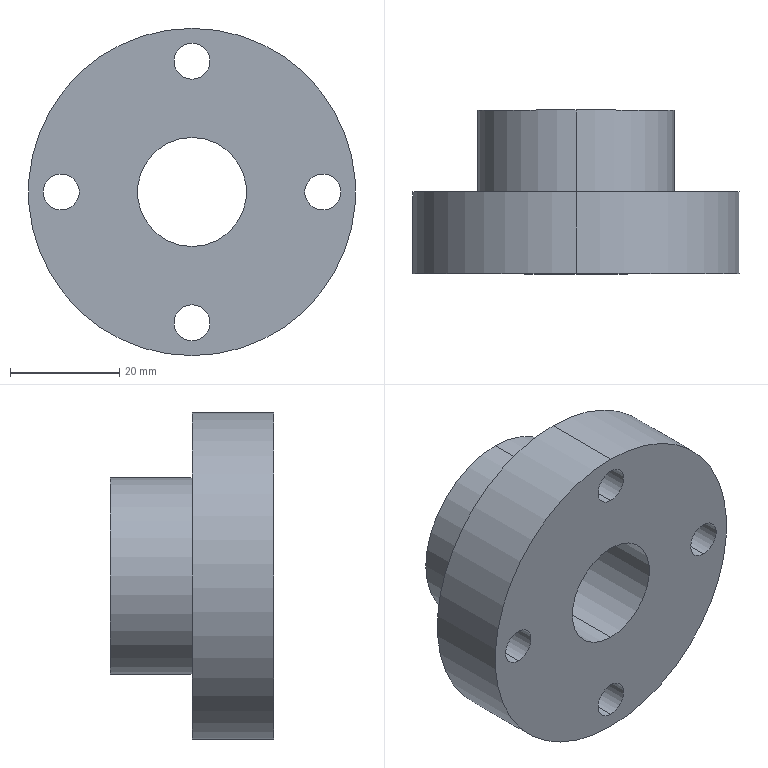Component | SolidWorks | OpticalAxisSeat1-1-1 | 1 solid | 29 faces | box 60 x 30 x 60 mm | volume 44996 mm3 | cylinder 22 | plane 7 | commonest cylinder face diameters 10 x8 6.6 x8 36 x2 60 x2 20 x2
build123d program:
from build123d import *

# Parameters (mm, degrees)
HOLE_SIZE_ACCORDING_TO_TYPE_1_OF_HEXAG_D           = 6.6
HOLE_SIZE_ACCORDING_TO_TYPE_1_OF_HEXAG_CBORE_D     = 10
HOLE_SIZE_ACCORDING_TO_TYPE_1_OF_HEXAG_CBORE_DEPTH = 6.8
CIRPATTERN1_COUNT                                  = 4


with BuildPart() as part:
    # Sketch1 → Revolve1 (revolve)
    with BuildSketch(Plane.XY, mode=Mode.PRIVATE) as revolve1_sk:
        Polygon((10, 1.22), (30, 1.22), (30, 16.22), (18, 16.22), (18, 31.22), (10, 31.22), align=None)
    revolve(revolve1_sk.sketch.rotate(Axis((0, 0, 0), (0, 1, 0)), 90), axis=Axis((0, 0, 0), (0, 1, 0)))

    # Hole Size _According to_ Type 1 of Hexag (through all)
    with Locations(Plane(origin=(24, 16.22, 0), x_dir=(0, 0, 1), z_dir=(0, 1, 0))):
        with Locations((0, 0)):
            hole_size_according_to_type_1_of_hexag = CounterBoreHole(HOLE_SIZE_ACCORDING_TO_TYPE_1_OF_HEXAG_D / 2, HOLE_SIZE_ACCORDING_TO_TYPE_1_OF_HEXAG_CBORE_D / 2, HOLE_SIZE_ACCORDING_TO_TYPE_1_OF_HEXAG_CBORE_DEPTH)

    # CirPattern1: Hole Size _According to_ Type 1 of Hexag ×4 about axis
    cirpattern1_axis = Axis((0, 0, 0), (0, 1, 0))
    for i in range(1, CIRPATTERN1_COUNT):
        add(hole_size_according_to_type_1_of_hexag.rotate(cirpattern1_axis, i * 360 / CIRPATTERN1_COUNT), mode=Mode.SUBTRACT)


solid = part.part

# Placed as in the assembly
solid = solid.moved(Location((-30.965, -1.22, 663.073), (0, 0, 0)))
STEP:
#1=CARTESIAN_POINT('',(-1.219,0.3228,24.964));
#2=VERTEX_POINT('',#1);
#3=CARTESIAN_POINT('',(-1.219,0.3228,25.357));
#4=VERTEX_POINT('',#3);
#5=CARTESIAN_POINT('',(-1.219,0.3228,25.16));
#6=DIRECTION('',(0.,1.,0.));
#7=DIRECTION('',(0.,0.,1.));
#8=AXIS2_PLACEMENT_3D('',#5,#6,#7);
#9=CIRCLE('',#8,0.1969);
#10=EDGE_CURVE('',#2,#4,#9,.T.);
#11=ORIENTED_EDGE('',*,*,#10,.F.);
#12=CARTESIAN_POINT('',(-1.219,0.5906,24.964));
#13=VERTEX_POINT('',#12);
#14=CARTESIAN_POINT('',(-1.219,0.5906,24.964));
#15=DIRECTION('',(0.,1.,0.));
#16=VECTOR('',#15,39.37);
#17=LINE('',#14,#16);
#18=EDGE_CURVE('',#2,#13,#17,.T.);
#19=ORIENTED_EDGE('',*,*,#18,.T.);
#20=CARTESIAN_POINT('',(-1.219,0.5906,25.357));
#21=VERTEX_POINT('',#20);
#22=CARTESIAN_POINT('',(-1.219,0.5906,25.16));
#23=DIRECTION('',(0.,1.,0.));
#24=DIRECTION('',(0.,0.,1.));
#25=AXIS2_PLACEMENT_3D('',#22,#23,#24);
#26=CIRCLE('',#25,0.1969);
#27=EDGE_CURVE('',#13,#21,#26,.T.);
#28=ORIENTED_EDGE('',*,*,#27,.T.);
#29=CARTESIAN_POINT('',(-1.219,0.5906,25.357));
#30=DIRECTION('',(0.,1.,0.));
#31=VECTOR('',#30,39.37);
#32=LINE('',#29,#31);
#33=EDGE_CURVE('',#4,#21,#32,.T.);
#34=ORIENTED_EDGE('',*,*,#33,.F.);
#35=EDGE_LOOP('',(#11,#19,#28,#34));
#36=FACE_OUTER_BOUND('',#35,.T.);
#37=CARTESIAN_POINT('',(-1.219,0.5906,25.16));
#38=DIRECTION('',(0.,1.,0.));
#39=DIRECTION('',(0.,0.,1.));
#40=AXIS2_PLACEMENT_3D('',#37,#38,#39);
#41=CYLINDRICAL_SURFACE('',#40,0.1969);
#42=ADVANCED_FACE('',(#36),#41,.F.);
#43=CARTESIAN_POINT('',(-1.219,-0.,25.03));
#44=VERTEX_POINT('',#43);
#45=CARTESIAN_POINT('',(-1.219,-0.,25.29));
#46=VERTEX_POINT('',#45);
#47=CARTESIAN_POINT('',(-1.219,-0.,25.16));
#48=DIRECTION('',(0.,1.,0.));
#49=DIRECTION('',(0.,0.,1.));
#50=AXIS2_PLACEMENT_3D('',#47,#48,#49);
#51=CIRCLE('',#50,0.1299);
#52=EDGE_CURVE('',#44,#46,#51,.T.);
#53=ORIENTED_EDGE('',*,*,#52,.F.);
#54=CARTESIAN_POINT('',(-1.219,0.3228,25.03));
#55=VERTEX_POINT('',#54);
#56=CARTESIAN_POINT('',(-1.219,0.5906,25.03));
#57=DIRECTION('',(0.,1.,0.));
#58=VECTOR('',#57,39.37);
#59=LINE('',#56,#58);
#60=EDGE_CURVE('',#44,#55,#59,.T.);
#61=ORIENTED_EDGE('',*,*,#60,.T.);
#62=CARTESIAN_POINT('',(-1.219,0.3228,25.29));
#63=VERTEX_POINT('',#62);
#64=CARTESIAN_POINT('',(-1.219,0.3228,25.16));
#65=DIRECTION('',(0.,1.,0.));
#66=DIRECTION('',(0.,0.,1.));
#67=AXIS2_PLACEMENT_3D('',#64,#65,#66);
#68=CIRCLE('',#67,0.1299);
#69=EDGE_CURVE('',#55,#63,#68,.T.);
#70=ORIENTED_EDGE('',*,*,#69,.T.);
#71=CARTESIAN_POINT('',(-1.219,0.5906,25.29));
#72=DIRECTION('',(0.,1.,0.));
#73=VECTOR('',#72,39.37);
#74=LINE('',#71,#73);
#75=EDGE_CURVE('',#46,#63,#74,.T.);
#76=ORIENTED_EDGE('',*,*,#75,.F.);
#77=EDGE_LOOP('',(#53,#61,#70,#76));
#78=FACE_OUTER_BOUND('',#77,.T.);
#79=CARTESIAN_POINT('',(-1.219,0.5906,25.16));
#80=DIRECTION('',(0.,1.,0.));
#81=DIRECTION('',(0.,0.,1.));
#82=AXIS2_PLACEMENT_3D('',#79,#80,#81);
#83=CYLINDRICAL_SURFACE('',#82,0.1299);
#84=ADVANCED_FACE('',(#78),#83,.F.);
#85=CARTESIAN_POINT('',(-2.164,0.3228,25.908));
#86=VERTEX_POINT('',#85);
#87=CARTESIAN_POINT('',(-2.164,0.3228,26.302));
#88=VERTEX_POINT('',#87);
#89=CARTESIAN_POINT('',(-2.164,0.3228,26.105));
#90=DIRECTION('',(0.,1.,0.));
#91=DIRECTION('',(0.,0.,1.));
#92=AXIS2_PLACEMENT_3D('',#89,#90,#91);
#93=CIRCLE('',#92,0.1969);
#94=EDGE_CURVE('',#86,#88,#93,.T.);
#95=ORIENTED_EDGE('',*,*,#94,.F.);
#96=CARTESIAN_POINT('',(-2.164,0.5906,25.908));
#97=VERTEX_POINT('',#96);
#98=CARTESIAN_POINT('',(-2.164,0.5906,25.908));
#99=DIRECTION('',(0.,1.,0.));
#100=VECTOR('',#99,39.37);
#101=LINE('',#98,#100);
#102=EDGE_CURVE('',#86,#97,#101,.T.);
#103=ORIENTED_EDGE('',*,*,#102,.T.);
#104=CARTESIAN_POINT('',(-2.164,0.5906,26.302));
#105=VERTEX_POINT('',#104);
#106=CARTESIAN_POINT('',(-2.164,0.5906,26.105));
#107=DIRECTION('',(0.,1.,0.));
#108=DIRECTION('',(0.,0.,1.));
#109=AXIS2_PLACEMENT_3D('',#106,#107,#108);
#110=CIRCLE('',#109,0.1969);
#111=EDGE_CURVE('',#97,#105,#110,.T.);
#112=ORIENTED_EDGE('',*,*,#111,.T.);
#113=CARTESIAN_POINT('',(-2.164,0.5906,26.302));
#114=DIRECTION('',(0.,1.,0.));
#115=VECTOR('',#114,39.37);
#116=LINE('',#113,#115);
#117=EDGE_CURVE('',#88,#105,#116,.T.);
#118=ORIENTED_EDGE('',*,*,#117,.F.);
#119=EDGE_LOOP('',(#95,#103,#112,#118));
#120=FACE_OUTER_BOUND('',#119,.T.);
#121=CARTESIAN_POINT('',(-2.164,0.5906,26.105));
#122=DIRECTION('',(0.,1.,0.));
#123=DIRECTION('',(0.,0.,1.));
#124=AXIS2_PLACEMENT_3D('',#121,#122,#123);
#125=CYLINDRICAL_SURFACE('',#124,0.1969);
#126=ADVANCED_FACE('',(#120),#125,.F.);
#127=CARTESIAN_POINT('',(-2.164,-0.,25.975));
#128=VERTEX_POINT('',#127);
#129=CARTESIAN_POINT('',(-2.164,-0.,26.235));
#130=VERTEX_POINT('',#129);
#131=CARTESIAN_POINT('',(-2.164,-0.,26.105));
#132=DIRECTION('',(0.,1.,0.));
#133=DIRECTION('',(0.,0.,1.));
#134=AXIS2_PLACEMENT_3D('',#131,#132,#133);
#135=CIRCLE('',#134,0.1299);
#136=EDGE_CURVE('',#128,#130,#135,.T.);
#137=ORIENTED_EDGE('',*,*,#136,.F.);
#138=CARTESIAN_POINT('',(-2.164,0.3228,25.975));
#139=VERTEX_POINT('',#138);
#140=CARTESIAN_POINT('',(-2.164,0.5906,25.975));
#141=DIRECTION('',(0.,1.,0.));
#142=VECTOR('',#141,39.37);
#143=LINE('',#140,#142);
#144=EDGE_CURVE('',#128,#139,#143,.T.);
#145=ORIENTED_EDGE('',*,*,#144,.T.);
#146=CARTESIAN_POINT('',(-2.164,0.3228,26.235));
#147=VERTEX_POINT('',#146);
#148=CARTESIAN_POINT('',(-2.164,0.3228,26.105));
#149=DIRECTION('',(0.,1.,0.));
#150=DIRECTION('',(0.,0.,1.));
#151=AXIS2_PLACEMENT_3D('',#148,#149,#150);
#152=CIRCLE('',#151,0.1299);
#153=EDGE_CURVE('',#139,#147,#152,.T.);
#154=ORIENTED_EDGE('',*,*,#153,.T.);
#155=CARTESIAN_POINT('',(-2.164,0.5906,26.235));
#156=DIRECTION('',(0.,1.,0.));
#157=VECTOR('',#156,39.37);
#158=LINE('',#155,#157);
#159=EDGE_CURVE('',#130,#147,#158,.T.);
#160=ORIENTED_EDGE('',*,*,#159,.F.);
#161=EDGE_LOOP('',(#137,#145,#154,#160));
#162=FACE_OUTER_BOUND('',#161,.T.);
#163=CARTESIAN_POINT('',(-2.164,0.5906,26.105));
#164=DIRECTION('',(0.,1.,0.));
#165=DIRECTION('',(0.,0.,1.));
#166=AXIS2_PLACEMENT_3D('',#163,#164,#165);
#167=CYLINDRICAL_SURFACE('',#166,0.1299);
#168=ADVANCED_FACE('',(#162),#167,.F.);
#169=CARTESIAN_POINT('',(-1.219,0.3228,26.853));
#170=VERTEX_POINT('',#169);
#171=CARTESIAN_POINT('',(-1.219,0.3228,27.247));
#172=VERTEX_POINT('',#171);
#173=CARTESIAN_POINT('',(-1.219,0.3228,27.05));
#174=DIRECTION('',(0.,1.,0.));
#175=DIRECTION('',(0.,0.,1.));
#176=AXIS2_PLACEMENT_3D('',#173,#174,#175);
#177=CIRCLE('',#176,0.1969);
#178=EDGE_CURVE('',#170,#172,#177,.T.);
#179=ORIENTED_EDGE('',*,*,#178,.F.);
#180=CARTESIAN_POINT('',(-1.219,0.5906,26.853));
#181=VERTEX_POINT('',#180);
#182=CARTESIAN_POINT('',(-1.219,0.5906,26.853));
#183=DIRECTION('',(0.,1.,0.));
#184=VECTOR('',#183,39.37);
#185=LINE('',#182,#184);
#186=EDGE_CURVE('',#170,#181,#185,.T.);
#187=ORIENTED_EDGE('',*,*,#186,.T.);
#188=CARTESIAN_POINT('',(-1.219,0.5906,27.247));
#189=VERTEX_POINT('',#188);
#190=CARTESIAN_POINT('',(-1.219,0.5906,27.05));
#191=DIRECTION('',(0.,1.,0.));
#192=DIRECTION('',(0.,0.,1.));
#193=AXIS2_PLACEMENT_3D('',#190,#191,#192);
#194=CIRCLE('',#193,0.1969);
#195=EDGE_CURVE('',#181,#189,#194,.T.);
#196=ORIENTED_EDGE('',*,*,#195,.T.);
#197=CARTESIAN_POINT('',(-1.219,0.5906,27.247));
#198=DIRECTION('',(0.,1.,0.));
#199=VECTOR('',#198,39.37);
#200=LINE('',#197,#199);
#201=EDGE_CURVE('',#172,#189,#200,.T.);
#202=ORIENTED_EDGE('',*,*,#201,.F.);
#203=EDGE_LOOP('',(#179,#187,#196,#202));
#204=FACE_OUTER_BOUND('',#203,.T.);
#205=CARTESIAN_POINT('',(-1.219,0.5906,27.05));
#206=DIRECTION('',(0.,1.,0.));
#207=DIRECTION('',(0.,0.,1.));
#208=AXIS2_PLACEMENT_3D('',#205,#206,#207);
#209=CYLINDRICAL_SURFACE('',#208,0.1969);
#210=ADVANCED_FACE('',(#204),#209,.F.);
#211=CARTESIAN_POINT('',(-1.219,-0.,26.92));
#212=VERTEX_POINT('',#211);
#213=CARTESIAN_POINT('',(-1.219,-0.,27.18));
#214=VERTEX_POINT('',#213);
#215=CARTESIAN_POINT('',(-1.219,-0.,27.05));
#216=DIRECTION('',(0.,1.,0.));
#217=DIRECTION('',(0.,0.,1.));
#218=AXIS2_PLACEMENT_3D('',#215,#216,#217);
#219=CIRCLE('',#218,0.1299);
#220=EDGE_CURVE('',#212,#214,#219,.T.);
#221=ORIENTED_EDGE('',*,*,#220,.F.);
#222=CARTESIAN_POINT('',(-1.219,0.3228,26.92));
#223=VERTEX_POINT('',#222);
#224=CARTESIAN_POINT('',(-1.219,0.5906,26.92));
#225=DIRECTION('',(0.,1.,0.));
#226=VECTOR('',#225,39.37);
#227=LINE('',#224,#226);
#228=EDGE_CURVE('',#212,#223,#227,.T.);
#229=ORIENTED_EDGE('',*,*,#228,.T.);
#230=CARTESIAN_POINT('',(-1.219,0.3228,27.18));
#231=VERTEX_POINT('',#230);
#232=CARTESIAN_POINT('',(-1.219,0.3228,27.05));
#233=DIRECTION('',(0.,1.,0.));
#234=DIRECTION('',(0.,0.,1.));
#235=AXIS2_PLACEMENT_3D('',#232,#233,#234);
#236=CIRCLE('',#235,0.1299);
#237=EDGE_CURVE('',#223,#231,#236,.T.);
#238=ORIENTED_EDGE('',*,*,#237,.T.);
#239=CARTESIAN_POINT('',(-1.219,0.5906,27.18));
#240=DIRECTION('',(0.,1.,0.));
#241=VECTOR('',#240,39.37);
#242=LINE('',#239,#241);
#243=EDGE_CURVE('',#214,#231,#242,.T.);
#244=ORIENTED_EDGE('',*,*,#243,.F.);
#245=EDGE_LOOP('',(#221,#229,#238,#244));
#246=FACE_OUTER_BOUND('',#245,.T.);
#247=CARTESIAN_POINT('',(-1.219,0.5906,27.05));
#248=DIRECTION('',(0.,1.,0.));
#249=DIRECTION('',(0.,0.,1.));
#250=AXIS2_PLACEMENT_3D('',#247,#248,#249);
#251=CYLINDRICAL_SURFACE('',#250,0.1299);
#252=ADVANCED_FACE('',(#246),#251,.F.);
#253=CARTESIAN_POINT('',(-0.2742,0.3228,25.908));
#254=VERTEX_POINT('',#253);
#255=CARTESIAN_POINT('',(-0.2742,0.3228,26.302));
#256=VERTEX_POINT('',#255);
#257=CARTESIAN_POINT('',(-0.2742,0.3228,26.105));
#258=DIRECTION('',(0.,1.,0.));
#259=DIRECTION('',(0.,0.,1.));
#260=AXIS2_PLACEMENT_3D('',#257,#258,#259);
#261=CIRCLE('',#260,0.1969);
#262=EDGE_CURVE('',#254,#256,#261,.T.);
#263=ORIENTED_EDGE('',*,*,#262,.F.);
#264=CARTESIAN_POINT('',(-0.2742,0.5906,25.908));
#265=VERTEX_POINT('',#264);
#266=CARTESIAN_POINT('',(-0.2742,0.5906,25.908));
#267=DIRECTION('',(0.,1.,0.));
#268=VECTOR('',#267,39.37);
#269=LINE('',#266,#268);
#270=EDGE_CURVE('',#254,#265,#269,.T.);
#271=ORIENTED_EDGE('',*,*,#270,.T.);
#272=CARTESIAN_POINT('',(-0.2742,0.5906,26.302));
#273=VERTEX_POINT('',#272);
#274=CARTESIAN_POINT('',(-0.2742,0.5906,26.105));
#275=DIRECTION('',(0.,1.,0.));
#276=DIRECTION('',(0.,0.,1.));
#277=AXIS2_PLACEMENT_3D('',#274,#275,#276);
#278=CIRCLE('',#277,0.1969);
#279=EDGE_CURVE('',#265,#273,#278,.T.);
#280=ORIENTED_EDGE('',*,*,#279,.T.);
#281=CARTESIAN_POINT('',(-0.2742,0.5906,26.302));
#282=DIRECTION('',(0.,1.,0.));
#283=VECTOR('',#282,39.37);
#284=LINE('',#281,#283);
#285=EDGE_CURVE('',#256,#273,#284,.T.);
#286=ORIENTED_EDGE('',*,*,#285,.F.);
#287=EDGE_LOOP('',(#263,#271,#280,#286));
#288=FACE_OUTER_BOUND('',#287,.T.);
#289=CARTESIAN_POINT('',(-0.2742,0.5906,26.105));
#290=DIRECTION('',(0.,1.,0.));
#291=DIRECTION('',(0.,0.,1.));
#292=AXIS2_PLACEMENT_3D('',#289,#290,#291);
#293=CYLINDRICAL_SURFACE('',#292,0.1969);
#294=ADVANCED_FACE('',(#288),#293,.F.);
#295=CARTESIAN_POINT('',(-0.2742,-0.,25.975));
#296=VERTEX_POINT('',#295);
#297=CARTESIAN_POINT('',(-0.2742,-0.,26.235));
#298=VERTEX_POINT('',#297);
#299=CARTESIAN_POINT('',(-0.2742,-0.,26.105));
#300=DIRECTION('',(0.,1.,0.));
#301=DIRECTION('',(0.,0.,1.));
#302=AXIS2_PLACEMENT_3D('',#299,#300,#301);
#303=CIRCLE('',#302,0.1299);
#304=EDGE_CURVE('',#296,#298,#303,.T.);
#305=ORIENTED_EDGE('',*,*,#304,.F.);
#306=CARTESIAN_POINT('',(-0.2742,0.3228,25.975));
#307=VERTEX_POINT('',#306);
#308=CARTESIAN_POINT('',(-0.2742,0.5906,25.975));
#309=DIRECTION('',(0.,1.,0.));
#310=VECTOR('',#309,39.37);
#311=LINE('',#308,#310);
#312=EDGE_CURVE('',#296,#307,#311,.T.);
#313=ORIENTED_EDGE('',*,*,#312,.T.);
#314=CARTESIAN_POINT('',(-0.2742,0.3228,26.235));
#315=VERTEX_POINT('',#314);
#316=CARTESIAN_POINT('',(-0.2742,0.3228,26.105));
#317=DIRECTION('',(0.,1.,0.));
#318=DIRECTION('',(0.,0.,1.));
#319=AXIS2_PLACEMENT_3D('',#316,#317,#318);
#320=CIRCLE('',#319,0.1299);
#321=EDGE_CURVE('',#307,#315,#320,.T.);
#322=ORIENTED_EDGE('',*,*,#321,.T.);
#323=CARTESIAN_POINT('',(-0.2742,0.5906,26.235));
#324=DIRECTION('',(0.,1.,0.));
#325=VECTOR('',#324,39.37);
#326=LINE('',#323,#325);
#327=EDGE_CURVE('',#298,#315,#326,.T.);
#328=ORIENTED_EDGE('',*,*,#327,.F.);
#329=EDGE_LOOP('',(#305,#313,#322,#328));
#330=FACE_OUTER_BOUND('',#329,.T.);
#331=CARTESIAN_POINT('',(-0.2742,0.5906,26.105));
#332=DIRECTION('',(0.,1.,0.));
#333=DIRECTION('',(0.,0.,1.));
#334=AXIS2_PLACEMENT_3D('',#331,#332,#333);
#335=CYLINDRICAL_SURFACE('',#334,0.1299);
#336=ADVANCED_FACE('',(#330),#335,.F.);
#337=CARTESIAN_POINT('',(-1.219,1.181,25.397));
#338=VERTEX_POINT('',#337);
#339=CARTESIAN_POINT('',(-1.219,1.181,26.814));
#340=VERTEX_POINT('',#339);
#341=CARTESIAN_POINT('',(-1.219,1.181,26.105));
#342=DIRECTION('',(0.,-1.,0.));
#343=DIRECTION('',(0.,0.,-1.));
#344=AXIS2_PLACEMENT_3D('',#341,#342,#343);
#345=CIRCLE('',#344,0.7087);
#346=EDGE_CURVE('',#338,#340,#345,.T.);
#347=ORIENTED_EDGE('',*,*,#346,.T.);
#348=CARTESIAN_POINT('',(-1.219,0.5906,26.814));
#349=VERTEX_POINT('',#348);
#350=CARTESIAN_POINT('',(-1.219,-0.04801,26.814));
#351=DIRECTION('',(0.,-1.,0.));
#352=VECTOR('',#351,39.37);
#353=LINE('',#350,#352);
#354=EDGE_CURVE('',#340,#349,#353,.T.);
#355=ORIENTED_EDGE('',*,*,#354,.T.);
#356=CARTESIAN_POINT('',(-1.219,0.5906,25.397));
#357=VERTEX_POINT('',#356);
#358=CARTESIAN_POINT('',(-1.219,0.5906,26.105));
#359=DIRECTION('',(0.,-1.,0.));
#360=DIRECTION('',(0.,0.,-1.));
#361=AXIS2_PLACEMENT_3D('',#358,#359,#360);
#362=CIRCLE('',#361,0.7087);
#363=EDGE_CURVE('',#357,#349,#362,.T.);
#364=ORIENTED_EDGE('',*,*,#363,.F.);
#365=CARTESIAN_POINT('',(-1.219,-0.04801,25.397));
#366=DIRECTION('',(0.,-1.,0.));
#367=VECTOR('',#366,39.37);
#368=LINE('',#365,#367);
#369=EDGE_CURVE('',#338,#357,#368,.T.);
#370=ORIENTED_EDGE('',*,*,#369,.F.);
#371=EDGE_LOOP('',(#347,#355,#364,#370));
#372=FACE_OUTER_BOUND('',#371,.T.);
#373=CARTESIAN_POINT('',(-1.219,-0.04801,26.105));
#374=DIRECTION('',(0.,-1.,0.));
#375=DIRECTION('',(0.,0.,-1.));
#376=AXIS2_PLACEMENT_3D('',#373,#374,#375);
#377=CYLINDRICAL_SURFACE('',#376,0.7087);
#378=ADVANCED_FACE('',(#372),#377,.T.);
#379=CARTESIAN_POINT('',(-1.219,0.5906,24.924));
#380=VERTEX_POINT('',#379);
#381=CARTESIAN_POINT('',(-1.219,0.5906,27.286));
#382=VERTEX_POINT('',#381);
#383=CARTESIAN_POINT('',(-1.219,0.5906,26.105));
#384=DIRECTION('',(0.,-1.,0.));
#385=DIRECTION('',(0.,0.,-1.));
#386=AXIS2_PLACEMENT_3D('',#383,#384,#385);
#387=CIRCLE('',#386,1.181);
#388=EDGE_CURVE('',#380,#382,#387,.T.);
#389=ORIENTED_EDGE('',*,*,#388,.T.);
#390=CARTESIAN_POINT('',(-1.219,-0.,27.286));
#391=VERTEX_POINT('',#390);
#392=CARTESIAN_POINT('',(-1.219,-0.04801,27.286));
#393=DIRECTION('',(0.,-1.,0.));
#394=VECTOR('',#393,39.37);
#395=LINE('',#392,#394);
#396=EDGE_CURVE('',#382,#391,#395,.T.);
#397=ORIENTED_EDGE('',*,*,#396,.T.);
#398=CARTESIAN_POINT('',(-1.219,-0.,24.924));
#399=VERTEX_POINT('',#398);
#400=CARTESIAN_POINT('',(-1.219,-0.,26.105));
#401=DIRECTION('',(0.,-1.,0.));
#402=DIRECTION('',(0.,0.,-1.));
#403=AXIS2_PLACEMENT_3D('',#400,#401,#402);
#404=CIRCLE('',#403,1.181);
#405=EDGE_CURVE('',#399,#391,#404,.T.);
#406=ORIENTED_EDGE('',*,*,#405,.F.);
#407=CARTESIAN_POINT('',(-1.219,-0.04801,24.924));
#408=DIRECTION('',(0.,-1.,0.));
#409=VECTOR('',#408,39.37);
#410=LINE('',#407,#409);
#411=EDGE_CURVE('',#380,#399,#410,.T.);
#412=ORIENTED_EDGE('',*,*,#411,.F.);
#413=EDGE_LOOP('',(#389,#397,#406,#412));
#414=FACE_OUTER_BOUND('',#413,.T.);
#415=CARTESIAN_POINT('',(-1.219,-0.04801,26.105));
#416=DIRECTION('',(0.,-1.,0.));
#417=DIRECTION('',(0.,0.,-1.));
#418=AXIS2_PLACEMENT_3D('',#415,#416,#417);
#419=CYLINDRICAL_SURFACE('',#418,1.181);
#420=ADVANCED_FACE('',(#414),#419,.T.);
#421=CARTESIAN_POINT('',(-1.219,1.181,26.499));
#422=VERTEX_POINT('',#421);
#423=CARTESIAN_POINT('',(-1.219,1.181,25.712));
#424=VERTEX_POINT('',#423);
#425=CARTESIAN_POINT('',(-1.219,1.181,26.105));
#426=DIRECTION('',(0.,-1.,0.));
#427=DIRECTION('',(0.,0.,-1.));
#428=AXIS2_PLACEMENT_3D('',#425,#426,#427);
#429=CIRCLE('',#428,0.3937);
#430=EDGE_CURVE('',#422,#424,#429,.T.);
#431=ORIENTED_EDGE('',*,*,#430,.F.);
#432=CARTESIAN_POINT('',(-1.219,-0.,26.499));
#433=VERTEX_POINT('',#432);
#434=CARTESIAN_POINT('',(-1.219,-0.04801,26.499));
#435=DIRECTION('',(0.,-1.,0.));
#436=VECTOR('',#435,39.37);
#437=LINE('',#434,#436);
#438=EDGE_CURVE('',#422,#433,#437,.T.);
#439=ORIENTED_EDGE('',*,*,#438,.T.);
#440=CARTESIAN_POINT('',(-1.219,-0.,25.712));
#441=VERTEX_POINT('',#440);
#442=CARTESIAN_POINT('',(-1.219,-0.,26.105));
#443=DIRECTION('',(0.,-1.,0.));
#444=DIRECTION('',(0.,0.,-1.));
#445=AXIS2_PLACEMENT_3D('',#442,#443,#444);
#446=CIRCLE('',#445,0.3937);
#447=EDGE_CURVE('',#433,#441,#446,.T.);
#448=ORIENTED_EDGE('',*,*,#447,.T.);
#449=CARTESIAN_POINT('',(-1.219,-0.04801,25.712));
#450=DIRECTION('',(0.,-1.,0.));
#451=VECTOR('',#450,39.37);
#452=LINE('',#449,#451);
#453=EDGE_CURVE('',#424,#441,#452,.T.);
#454=ORIENTED_EDGE('',*,*,#453,.F.);
#455=EDGE_LOOP('',(#431,#439,#448,#454));
#456=FACE_OUTER_BOUND('',#455,.T.);
#457=CARTESIAN_POINT('',(-1.219,-0.04801,26.105));
#458=DIRECTION('',(0.,-1.,0.));
#459=DIRECTION('',(0.,0.,-1.));
#460=AXIS2_PLACEMENT_3D('',#457,#458,#459);
#461=CYLINDRICAL_SURFACE('',#460,0.3937);
#462=ADVANCED_FACE('',(#456),#461,.F.);
#463=ORIENTED_EDGE('',*,*,#438,.F.);
#464=CARTESIAN_POINT('',(-1.219,1.181,26.105));
#465=DIRECTION('',(0.,-1.,0.));
#466=DIRECTION('',(0.,0.,-1.));
#467=AXIS2_PLACEMENT_3D('',#464,#465,#466);
#468=CIRCLE('',#467,0.3937);
#469=EDGE_CURVE('',#424,#422,#468,.T.);
#470=ORIENTED_EDGE('',*,*,#469,.F.);
#471=ORIENTED_EDGE('',*,*,#453,.T.);
#472=CARTESIAN_POINT('',(-1.219,-0.,26.105));
#473=DIRECTION('',(0.,-1.,0.));
#474=DIRECTION('',(0.,0.,-1.));
#475=AXIS2_PLACEMENT_3D('',#472,#473,#474);
#476=CIRCLE('',#475,0.3937);
#477=EDGE_CURVE('',#441,#433,#476,.T.);
#478=ORIENTED_EDGE('',*,*,#477,.T.);
#479=EDGE_LOOP('',(#463,#470,#471,#478));
#480=FACE_OUTER_BOUND('',#479,.T.);
#481=CARTESIAN_POINT('',(-1.219,-0.04801,26.105));
#482=DIRECTION('',(0.,-1.,0.));
#483=DIRECTION('',(0.,0.,-1.));
#484=AXIS2_PLACEMENT_3D('',#481,#482,#483);
#485=CYLINDRICAL_SURFACE('',#484,0.3937);
#486=ADVANCED_FACE('',(#480),#485,.F.);
#487=CARTESIAN_POINT('',(-1.219,-0.,25.16));
#488=DIRECTION('',(0.,1.,0.));
#489=DIRECTION('',(0.,0.,1.));
#490=AXIS2_PLACEMENT_3D('',#487,#488,#489);
#491=CIRCLE('',#490,0.1299);
#492=EDGE_CURVE('',#46,#44,#491,.T.);
#493=ORIENTED_EDGE('',*,*,#492,.T.);
#494=ORIENTED_EDGE('',*,*,#52,.T.);
#495=EDGE_LOOP('',(#493,#494));
#496=FACE_BOUND('',#495,.T.);
#497=CARTESIAN_POINT('',(-2.164,-0.,26.105));
#498=DIRECTION('',(0.,1.,0.));
#499=DIRECTION('',(0.,0.,1.));
#500=AXIS2_PLACEMENT_3D('',#497,#498,#499);
#501=CIRCLE('',#500,0.1299);
#502=EDGE_CURVE('',#130,#128,#501,.T.);
#503=ORIENTED_EDGE('',*,*,#502,.T.);
#504=ORIENTED_EDGE('',*,*,#136,.T.);
#505=EDGE_LOOP('',(#503,#504));
#506=FACE_BOUND('',#505,.T.);
#507=CARTESIAN_POINT('',(-1.219,-0.,27.05));
#508=DIRECTION('',(0.,1.,0.));
#509=DIRECTION('',(0.,0.,1.));
#510=AXIS2_PLACEMENT_3D('',#507,#508,#509);
#511=CIRCLE('',#510,0.1299);
#512=EDGE_CURVE('',#214,#212,#511,.T.);
#513=ORIENTED_EDGE('',*,*,#512,.T.);
#514=ORIENTED_EDGE('',*,*,#220,.T.);
#515=EDGE_LOOP('',(#513,#514));
#516=FACE_BOUND('',#515,.T.);
#517=CARTESIAN_POINT('',(-0.2742,-0.,26.105));
#518=DIRECTION('',(0.,1.,0.));
#519=DIRECTION('',(0.,0.,1.));
#520=AXIS2_PLACEMENT_3D('',#517,#518,#519);
#521=CIRCLE('',#520,0.1299);
#522=EDGE_CURVE('',#298,#296,#521,.T.);
#523=ORIENTED_EDGE('',*,*,#522,.T.);
#524=ORIENTED_EDGE('',*,*,#304,.T.);
#525=EDGE_LOOP('',(#523,#524));
#526=FACE_BOUND('',#525,.T.);
#527=ORIENTED_EDGE('',*,*,#405,.T.);
#528=CARTESIAN_POINT('',(-1.219,-0.,26.105));
#529=DIRECTION('',(0.,-1.,0.));
#530=DIRECTION('',(0.,0.,-1.));
#531=AXIS2_PLACEMENT_3D('',#528,#529,#530);
#532=CIRCLE('',#531,1.181);
#533=EDGE_CURVE('',#391,#399,#532,.T.);
#534=ORIENTED_EDGE('',*,*,#533,.T.);
#535=EDGE_LOOP('',(#527,#534));
#536=FACE_OUTER_BOUND('',#535,.T.);
#537=ORIENTED_EDGE('',*,*,#477,.F.);
#538=ORIENTED_EDGE('',*,*,#447,.F.);
#539=EDGE_LOOP('',(#537,#538));
#540=FACE_BOUND('',#539,.T.);
#541=CARTESIAN_POINT('',(-0.8254,-0.,26.105));
#542=DIRECTION('',(0.,-1.,0.));
#543=DIRECTION('',(0.,0.,-1.));
#544=AXIS2_PLACEMENT_3D('',#541,#542,#543);
#545=PLANE('',#544);
#546=ADVANCED_FACE('',(#496,#506,#516,#526,#536,#540),#545,.T.);
#547=ORIENTED_EDGE('',*,*,#396,.F.);
#548=CARTESIAN_POINT('',(-1.219,0.5906,26.105));
#549=DIRECTION('',(0.,-1.,0.));
#550=DIRECTION('',(0.,0.,-1.));
#551=AXIS2_PLACEMENT_3D('',#548,#549,#550);
#552=CIRCLE('',#551,1.181);
#553=EDGE_CURVE('',#382,#380,#552,.T.);
#554=ORIENTED_EDGE('',*,*,#553,.T.);
#555=ORIENTED_EDGE('',*,*,#411,.T.);
#556=ORIENTED_EDGE('',*,*,#533,.F.);
#557=EDGE_LOOP('',(#547,#554,#555,#556));
#558=FACE_OUTER_BOUND('',#557,.T.);
#559=CARTESIAN_POINT('',(-1.219,-0.04801,26.105));
#560=DIRECTION('',(0.,-1.,0.));
#561=DIRECTION('',(0.,0.,-1.));
#562=AXIS2_PLACEMENT_3D('',#559,#560,#561);
#563=CYLINDRICAL_SURFACE('',#562,1.181);
#564=ADVANCED_FACE('',(#558),#563,.T.);
#565=CARTESIAN_POINT('',(-1.219,0.5906,25.16));
#566=DIRECTION('',(0.,1.,0.));
#567=DIRECTION('',(0.,0.,1.));
#568=AXIS2_PLACEMENT_3D('',#565,#566,#567);
#569=CIRCLE('',#568,0.1969);
#570=EDGE_CURVE('',#21,#13,#569,.T.);
#571=ORIENTED_EDGE('',*,*,#570,.F.);
#572=ORIENTED_EDGE('',*,*,#27,.F.);
#573=EDGE_LOOP('',(#571,#572));
#574=FACE_BOUND('',#573,.T.);
#575=CARTESIAN_POINT('',(-2.164,0.5906,26.105));
#576=DIRECTION('',(0.,1.,0.));
#577=DIRECTION('',(0.,0.,1.));
#578=AXIS2_PLACEMENT_3D('',#575,#576,#577);
#579=CIRCLE('',#578,0.1969);
#580=EDGE_CURVE('',#105,#97,#579,.T.);
#581=ORIENTED_EDGE('',*,*,#580,.F.);
#582=ORIENTED_EDGE('',*,*,#111,.F.);
#583=EDGE_LOOP('',(#581,#582));
#584=FACE_BOUND('',#583,.T.);
#585=CARTESIAN_POINT('',(-1.219,0.5906,27.05));
#586=DIRECTION('',(0.,1.,0.));
#587=DIRECTION('',(0.,0.,1.));
#588=AXIS2_PLACEMENT_3D('',#585,#586,#587);
#589=CIRCLE('',#588,0.1969);
#590=EDGE_CURVE('',#189,#181,#589,.T.);
#591=ORIENTED_EDGE('',*,*,#590,.F.);
#592=ORIENTED_EDGE('',*,*,#195,.F.);
#593=EDGE_LOOP('',(#591,#592));
#594=FACE_BOUND('',#593,.T.);
#595=CARTESIAN_POINT('',(-0.2742,0.5906,26.105));
#596=DIRECTION('',(0.,1.,0.));
#597=DIRECTION('',(0.,0.,1.));
#598=AXIS2_PLACEMENT_3D('',#595,#596,#597);
#599=CIRCLE('',#598,0.1969);
#600=EDGE_CURVE('',#273,#265,#599,.T.);
#601=ORIENTED_EDGE('',*,*,#600,.F.);
#602=ORIENTED_EDGE('',*,*,#279,.F.);
#603=EDGE_LOOP('',(#601,#602));
#604=FACE_BOUND('',#603,.T.);
#605=ORIENTED_EDGE('',*,*,#363,.T.);
#606=CARTESIAN_POINT('',(-1.219,0.5906,26.105));
#607=DIRECTION('',(0.,-1.,0.));
#608=DIRECTION('',(0.,0.,-1.));
#609=AXIS2_PLACEMENT_3D('',#606,#607,#608);
#610=CIRCLE('',#609,0.7087);
#611=EDGE_CURVE('',#349,#357,#610,.T.);
#612=ORIENTED_EDGE('',*,*,#611,.T.);
#613=EDGE_LOOP('',(#605,#612));
#614=FACE_BOUND('',#613,.T.);
#615=ORIENTED_EDGE('',*,*,#388,.F.);
#616=ORIENTED_EDGE('',*,*,#553,.F.);
#617=EDGE_LOOP('',(#615,#616));
#618=FACE_OUTER_BOUND('',#617,.T.);
#619=CARTESIAN_POINT('',(-0.03799,0.5906,26.105));
#620=DIRECTION('',(0.,1.,0.));
#621=DIRECTION('',(0.,0.,1.));
#622=AXIS2_PLACEMENT_3D('',#619,#620,#621);
#623=PLANE('',#622);
#624=ADVANCED_FACE('',(#574,#584,#594,#604,#614,#618),#623,.T.);
#625=ORIENTED_EDGE('',*,*,#354,.F.);
#626=CARTESIAN_POINT('',(-1.219,1.181,26.105));
#627=DIRECTION('',(0.,-1.,0.));
#628=DIRECTION('',(0.,0.,-1.));
#629=AXIS2_PLACEMENT_3D('',#626,#627,#628);
#630=CIRCLE('',#629,0.7087);
#631=EDGE_CURVE('',#340,#338,#630,.T.);
#632=ORIENTED_EDGE('',*,*,#631,.T.);
#633=ORIENTED_EDGE('',*,*,#369,.T.);
#634=ORIENTED_EDGE('',*,*,#611,.F.);
#635=EDGE_LOOP('',(#625,#632,#633,#634));
#636=FACE_OUTER_BOUND('',#635,.T.);
#637=CARTESIAN_POINT('',(-1.219,-0.04801,26.105));
#638=DIRECTION('',(0.,-1.,0.));
#639=DIRECTION('',(0.,0.,-1.));
#640=AXIS2_PLACEMENT_3D('',#637,#638,#639);
#641=CYLINDRICAL_SURFACE('',#640,0.7087);
#642=ADVANCED_FACE('',(#636),#641,.T.);
#643=ORIENTED_EDGE('',*,*,#469,.T.);
#644=ORIENTED_EDGE('',*,*,#430,.T.);
#645=EDGE_LOOP('',(#643,#644));
#646=FACE_BOUND('',#645,.T.);
#647=ORIENTED_EDGE('',*,*,#346,.F.);
#648=ORIENTED_EDGE('',*,*,#631,.F.);
#649=EDGE_LOOP('',(#647,#648));
#650=FACE_OUTER_BOUND('',#649,.T.);
#651=CARTESIAN_POINT('',(-0.5104,1.181,26.105));
#652=DIRECTION('',(0.,1.,0.));
#653=DIRECTION('',(0.,0.,1.));
#654=AXIS2_PLACEMENT_3D('',#651,#652,#653);
#655=PLANE('',#654);
#656=ADVANCED_FACE('',(#646,#650),#655,.T.);
#657=ORIENTED_EDGE('',*,*,#312,.F.);
#658=ORIENTED_EDGE('',*,*,#522,.F.);
#659=ORIENTED_EDGE('',*,*,#327,.T.);
#660=CARTESIAN_POINT('',(-0.2742,0.3228,26.105));
#661=DIRECTION('',(0.,1.,0.));
#662=DIRECTION('',(0.,0.,1.));
#663=AXIS2_PLACEMENT_3D('',#660,#661,#662);
#664=CIRCLE('',#663,0.1299);
#665=EDGE_CURVE('',#315,#307,#664,.T.);
#666=ORIENTED_EDGE('',*,*,#665,.T.);
#667=EDGE_LOOP('',(#657,#658,#659,#666));
#668=FACE_OUTER_BOUND('',#667,.T.);
#669=CARTESIAN_POINT('',(-0.2742,0.5906,26.105));
#670=DIRECTION('',(0.,1.,0.));
#671=DIRECTION('',(0.,0.,1.));
#672=AXIS2_PLACEMENT_3D('',#669,#670,#671);
#673=CYLINDRICAL_SURFACE('',#672,0.1299);
#674=ADVANCED_FACE('',(#668),#673,.F.);
#675=ORIENTED_EDGE('',*,*,#665,.F.);
#676=ORIENTED_EDGE('',*,*,#321,.F.);
#677=EDGE_LOOP('',(#675,#676));
#678=FACE_BOUND('',#677,.T.);
#679=CARTESIAN_POINT('',(-0.2742,0.3228,26.105));
#680=DIRECTION('',(0.,1.,0.));
#681=DIRECTION('',(0.,0.,1.));
#682=AXIS2_PLACEMENT_3D('',#679,#680,#681);
#683=CIRCLE('',#682,0.1969);
#684=EDGE_CURVE('',#256,#254,#683,.T.);
#685=ORIENTED_EDGE('',*,*,#684,.T.);
#686=ORIENTED_EDGE('',*,*,#262,.T.);
#687=EDGE_LOOP('',(#685,#686));
#688=FACE_OUTER_BOUND('',#687,.T.);
#689=CARTESIAN_POINT('',(-0.1443,0.3228,26.105));
#690=DIRECTION('',(0.,-1.,0.));
#691=DIRECTION('',(0.,0.,-1.));
#692=AXIS2_PLACEMENT_3D('',#689,#690,#691);
#693=PLANE('',#692);
#694=ADVANCED_FACE('',(#678,#688),#693,.F.);
#695=ORIENTED_EDGE('',*,*,#270,.F.);
#696=ORIENTED_EDGE('',*,*,#684,.F.);
#697=ORIENTED_EDGE('',*,*,#285,.T.);
#698=ORIENTED_EDGE('',*,*,#600,.T.);
#699=EDGE_LOOP('',(#695,#696,#697,#698));
#700=FACE_OUTER_BOUND('',#699,.T.);
#701=CARTESIAN_POINT('',(-0.2742,0.5906,26.105));
#702=DIRECTION('',(0.,1.,0.));
#703=DIRECTION('',(0.,0.,1.));
#704=AXIS2_PLACEMENT_3D('',#701,#702,#703);
#705=CYLINDRICAL_SURFACE('',#704,0.1969);
#706=ADVANCED_FACE('',(#700),#705,.F.);
#707=ORIENTED_EDGE('',*,*,#228,.F.);
#708=ORIENTED_EDGE('',*,*,#512,.F.);
#709=ORIENTED_EDGE('',*,*,#243,.T.);
#710=CARTESIAN_POINT('',(-1.219,0.3228,27.05));
#711=DIRECTION('',(0.,1.,0.));
#712=DIRECTION('',(0.,0.,1.));
#713=AXIS2_PLACEMENT_3D('',#710,#711,#712);
#714=CIRCLE('',#713,0.1299);
#715=EDGE_CURVE('',#231,#223,#714,.T.);
#716=ORIENTED_EDGE('',*,*,#715,.T.);
#717=EDGE_LOOP('',(#707,#708,#709,#716));
#718=FACE_OUTER_BOUND('',#717,.T.);
#719=CARTESIAN_POINT('',(-1.219,0.5906,27.05));
#720=DIRECTION('',(0.,1.,0.));
#721=DIRECTION('',(0.,0.,1.));
#722=AXIS2_PLACEMENT_3D('',#719,#720,#721);
#723=CYLINDRICAL_SURFACE('',#722,0.1299);
#724=ADVANCED_FACE('',(#718),#723,.F.);
#725=ORIENTED_EDGE('',*,*,#715,.F.);
#726=ORIENTED_EDGE('',*,*,#237,.F.);
#727=EDGE_LOOP('',(#725,#726));
#728=FACE_BOUND('',#727,.T.);
#729=CARTESIAN_POINT('',(-1.219,0.3228,27.05));
#730=DIRECTION('',(0.,1.,0.));
#731=DIRECTION('',(0.,0.,1.));
#732=AXIS2_PLACEMENT_3D('',#729,#730,#731);
#733=CIRCLE('',#732,0.1969);
#734=EDGE_CURVE('',#172,#170,#733,.T.);
#735=ORIENTED_EDGE('',*,*,#734,.T.);
#736=ORIENTED_EDGE('',*,*,#178,.T.);
#737=EDGE_LOOP('',(#735,#736));
#738=FACE_OUTER_BOUND('',#737,.T.);
#739=CARTESIAN_POINT('',(-1.089,0.3228,27.05));
#740=DIRECTION('',(0.,-1.,0.));
#741=DIRECTION('',(0.,0.,-1.));
#742=AXIS2_PLACEMENT_3D('',#739,#740,#741);
#743=PLANE('',#742);
#744=ADVANCED_FACE('',(#728,#738),#743,.F.);
#745=ORIENTED_EDGE('',*,*,#186,.F.);
#746=ORIENTED_EDGE('',*,*,#734,.F.);
#747=ORIENTED_EDGE('',*,*,#201,.T.);
#748=ORIENTED_EDGE('',*,*,#590,.T.);
#749=EDGE_LOOP('',(#745,#746,#747,#748));
#750=FACE_OUTER_BOUND('',#749,.T.);
#751=CARTESIAN_POINT('',(-1.219,0.5906,27.05));
#752=DIRECTION('',(0.,1.,0.));
#753=DIRECTION('',(0.,0.,1.));
#754=AXIS2_PLACEMENT_3D('',#751,#752,#753);
#755=CYLINDRICAL_SURFACE('',#754,0.1969);
#756=ADVANCED_FACE('',(#750),#755,.F.);
#757=ORIENTED_EDGE('',*,*,#144,.F.);
#758=ORIENTED_EDGE('',*,*,#502,.F.);
#759=ORIENTED_EDGE('',*,*,#159,.T.);
#760=CARTESIAN_POINT('',(-2.164,0.3228,26.105));
#761=DIRECTION('',(0.,1.,0.));
#762=DIRECTION('',(0.,0.,1.));
#763=AXIS2_PLACEMENT_3D('',#760,#761,#762);
#764=CIRCLE('',#763,0.1299);
#765=EDGE_CURVE('',#147,#139,#764,.T.);
#766=ORIENTED_EDGE('',*,*,#765,.T.);
#767=EDGE_LOOP('',(#757,#758,#759,#766));
#768=FACE_OUTER_BOUND('',#767,.T.);
#769=CARTESIAN_POINT('',(-2.164,0.5906,26.105));
#770=DIRECTION('',(0.,1.,0.));
#771=DIRECTION('',(0.,0.,1.));
#772=AXIS2_PLACEMENT_3D('',#769,#770,#771);
#773=CYLINDRICAL_SURFACE('',#772,0.1299);
#774=ADVANCED_FACE('',(#768),#773,.F.);
#775=ORIENTED_EDGE('',*,*,#765,.F.);
#776=ORIENTED_EDGE('',*,*,#153,.F.);
#777=EDGE_LOOP('',(#775,#776));
#778=FACE_BOUND('',#777,.T.);
#779=CARTESIAN_POINT('',(-2.164,0.3228,26.105));
#780=DIRECTION('',(0.,1.,0.));
#781=DIRECTION('',(0.,0.,1.));
#782=AXIS2_PLACEMENT_3D('',#779,#780,#781);
#783=CIRCLE('',#782,0.1969);
#784=EDGE_CURVE('',#88,#86,#783,.T.);
#785=ORIENTED_EDGE('',*,*,#784,.T.);
#786=ORIENTED_EDGE('',*,*,#94,.T.);
#787=EDGE_LOOP('',(#785,#786));
#788=FACE_OUTER_BOUND('',#787,.T.);
#789=CARTESIAN_POINT('',(-2.034,0.3228,26.105));
#790=DIRECTION('',(0.,-1.,0.));
#791=DIRECTION('',(0.,0.,-1.));
#792=AXIS2_PLACEMENT_3D('',#789,#790,#791);
#793=PLANE('',#792);
#794=ADVANCED_FACE('',(#778,#788),#793,.F.);
#795=ORIENTED_EDGE('',*,*,#102,.F.);
#796=ORIENTED_EDGE('',*,*,#784,.F.);
#797=ORIENTED_EDGE('',*,*,#117,.T.);
#798=ORIENTED_EDGE('',*,*,#580,.T.);
#799=EDGE_LOOP('',(#795,#796,#797,#798));
#800=FACE_OUTER_BOUND('',#799,.T.);
#801=CARTESIAN_POINT('',(-2.164,0.5906,26.105));
#802=DIRECTION('',(0.,1.,0.));
#803=DIRECTION('',(0.,0.,1.));
#804=AXIS2_PLACEMENT_3D('',#801,#802,#803);
#805=CYLINDRICAL_SURFACE('',#804,0.1969);
#806=ADVANCED_FACE('',(#800),#805,.F.);
#807=ORIENTED_EDGE('',*,*,#60,.F.);
#808=ORIENTED_EDGE('',*,*,#492,.F.);
#809=ORIENTED_EDGE('',*,*,#75,.T.);
#810=CARTESIAN_POINT('',(-1.219,0.3228,25.16));
#811=DIRECTION('',(0.,1.,0.));
#812=DIRECTION('',(0.,0.,1.));
#813=AXIS2_PLACEMENT_3D('',#810,#811,#812);
#814=CIRCLE('',#813,0.1299);
#815=EDGE_CURVE('',#63,#55,#814,.T.);
#816=ORIENTED_EDGE('',*,*,#815,.T.);
#817=EDGE_LOOP('',(#807,#808,#809,#816));
#818=FACE_OUTER_BOUND('',#817,.T.);
#819=CARTESIAN_POINT('',(-1.219,0.5906,25.16));
#820=DIRECTION('',(0.,1.,0.));
#821=DIRECTION('',(0.,0.,1.));
#822=AXIS2_PLACEMENT_3D('',#819,#820,#821);
#823=CYLINDRICAL_SURFACE('',#822,0.1299);
#824=ADVANCED_FACE('',(#818),#823,.F.);
#825=ORIENTED_EDGE('',*,*,#815,.F.);
#826=ORIENTED_EDGE('',*,*,#69,.F.);
#827=EDGE_LOOP('',(#825,#826));
#828=FACE_BOUND('',#827,.T.);
#829=CARTESIAN_POINT('',(-1.219,0.3228,25.16));
#830=DIRECTION('',(0.,1.,0.));
#831=DIRECTION('',(0.,0.,1.));
#832=AXIS2_PLACEMENT_3D('',#829,#830,#831);
#833=CIRCLE('',#832,0.1969);
#834=EDGE_CURVE('',#4,#2,#833,.T.);
#835=ORIENTED_EDGE('',*,*,#834,.T.);
#836=ORIENTED_EDGE('',*,*,#10,.T.);
#837=EDGE_LOOP('',(#835,#836));
#838=FACE_OUTER_BOUND('',#837,.T.);
#839=CARTESIAN_POINT('',(-1.089,0.3228,25.16));
#840=DIRECTION('',(0.,-1.,0.));
#841=DIRECTION('',(0.,0.,-1.));
#842=AXIS2_PLACEMENT_3D('',#839,#840,#841);
#843=PLANE('',#842);
#844=ADVANCED_FACE('',(#828,#838),#843,.F.);
#845=ORIENTED_EDGE('',*,*,#18,.F.);
#846=ORIENTED_EDGE('',*,*,#834,.F.);
#847=ORIENTED_EDGE('',*,*,#33,.T.);
#848=ORIENTED_EDGE('',*,*,#570,.T.);
#849=EDGE_LOOP('',(#845,#846,#847,#848));
#850=FACE_OUTER_BOUND('',#849,.T.);
#851=CARTESIAN_POINT('',(-1.219,0.5906,25.16));
#852=DIRECTION('',(0.,1.,0.));
#853=DIRECTION('',(0.,0.,1.));
#854=AXIS2_PLACEMENT_3D('',#851,#852,#853);
#855=CYLINDRICAL_SURFACE('',#854,0.1969);
#856=ADVANCED_FACE('',(#850),#855,.F.);
#857=CLOSED_SHELL('',(#42,#84,#126,#168,#210,#252,#294,#336,#378,#420,#462,#486,#546,#564,#624,#642,#656,#674,#694,#706,#724,#744,#756,#774,#794,#806,#824,#844,#856));
#858=MANIFOLD_SOLID_BREP('',#857);
#859=CARTESIAN_POINT('',(0.,0.,0.));
#860=DIRECTION('',(0.,0.,1.));
#861=DIRECTION('',(1.,0.,0.));
#862=AXIS2_PLACEMENT_3D('',#859,#860,#861);
#863=(LENGTH_UNIT()NAMED_UNIT(*)SI_UNIT($,.METRE.));
#864=LENGTH_MEASURE_WITH_UNIT(LENGTH_MEASURE(0.0254),#863);
#865=DIMENSIONAL_EXPONENTS(1.,0.,0.,0.,0.,0.,0.);
#866=(CONVERSION_BASED_UNIT('',#864)LENGTH_UNIT()NAMED_UNIT(#865));
#867=UNCERTAINTY_MEASURE_WITH_UNIT(LENGTH_MEASURE(0.00001),#866,'','');
#868=(NAMED_UNIT(*)PLANE_ANGLE_UNIT()SI_UNIT($,.RADIAN.));
#869=(NAMED_UNIT(*)SI_UNIT($,.STERADIAN.)SOLID_ANGLE_UNIT());
#870=(GEOMETRIC_REPRESENTATION_CONTEXT(3)GLOBAL_UNCERTAINTY_ASSIGNED_CONTEXT((#867))GLOBAL_UNIT_ASSIGNED_CONTEXT((#866,#868,#869))REPRESENTATION_CONTEXT('',''));
#871=ADVANCED_BREP_SHAPE_REPRESENTATION('',(#858,#862),#870);
#872=COLOUR_RGB('',0.7922,0.8196,0.9333);
#873=FILL_AREA_STYLE_COLOUR('',#872);
#874=FILL_AREA_STYLE('',(#873));
#875=SURFACE_STYLE_FILL_AREA(#874);
#876=SURFACE_SIDE_STYLE('',(#875));
#877=SURFACE_STYLE_USAGE(.BOTH.,#876);
#878=PRESENTATION_STYLE_ASSIGNMENT((#877));
#879=STYLED_ITEM('',(#878),#858);
#880=(LENGTH_UNIT()NAMED_UNIT(*)SI_UNIT($,.METRE.));
#881=LENGTH_MEASURE_WITH_UNIT(LENGTH_MEASURE(0.0254),#880);
#882=DIMENSIONAL_EXPONENTS(1.,0.,0.,0.,0.,0.,0.);
#883=(CONVERSION_BASED_UNIT('',#881)LENGTH_UNIT()NAMED_UNIT(#882));
#884=UNCERTAINTY_MEASURE_WITH_UNIT(LENGTH_MEASURE(0.00001),#883,'','');
#885=(NAMED_UNIT(*)PLANE_ANGLE_UNIT()SI_UNIT($,.RADIAN.));
#886=(NAMED_UNIT(*)SI_UNIT($,.STERADIAN.)SOLID_ANGLE_UNIT());
#887=(GEOMETRIC_REPRESENTATION_CONTEXT(3)GLOBAL_UNCERTAINTY_ASSIGNED_CONTEXT((#884))GLOBAL_UNIT_ASSIGNED_CONTEXT((#883,#885,#886))REPRESENTATION_CONTEXT('',''));
#888=MECHANICAL_DESIGN_GEOMETRIC_PRESENTATION_REPRESENTATION('',(#879),#887);
#889=PRESENTATION_LAYER_ASSIGNMENT('','',(#879));